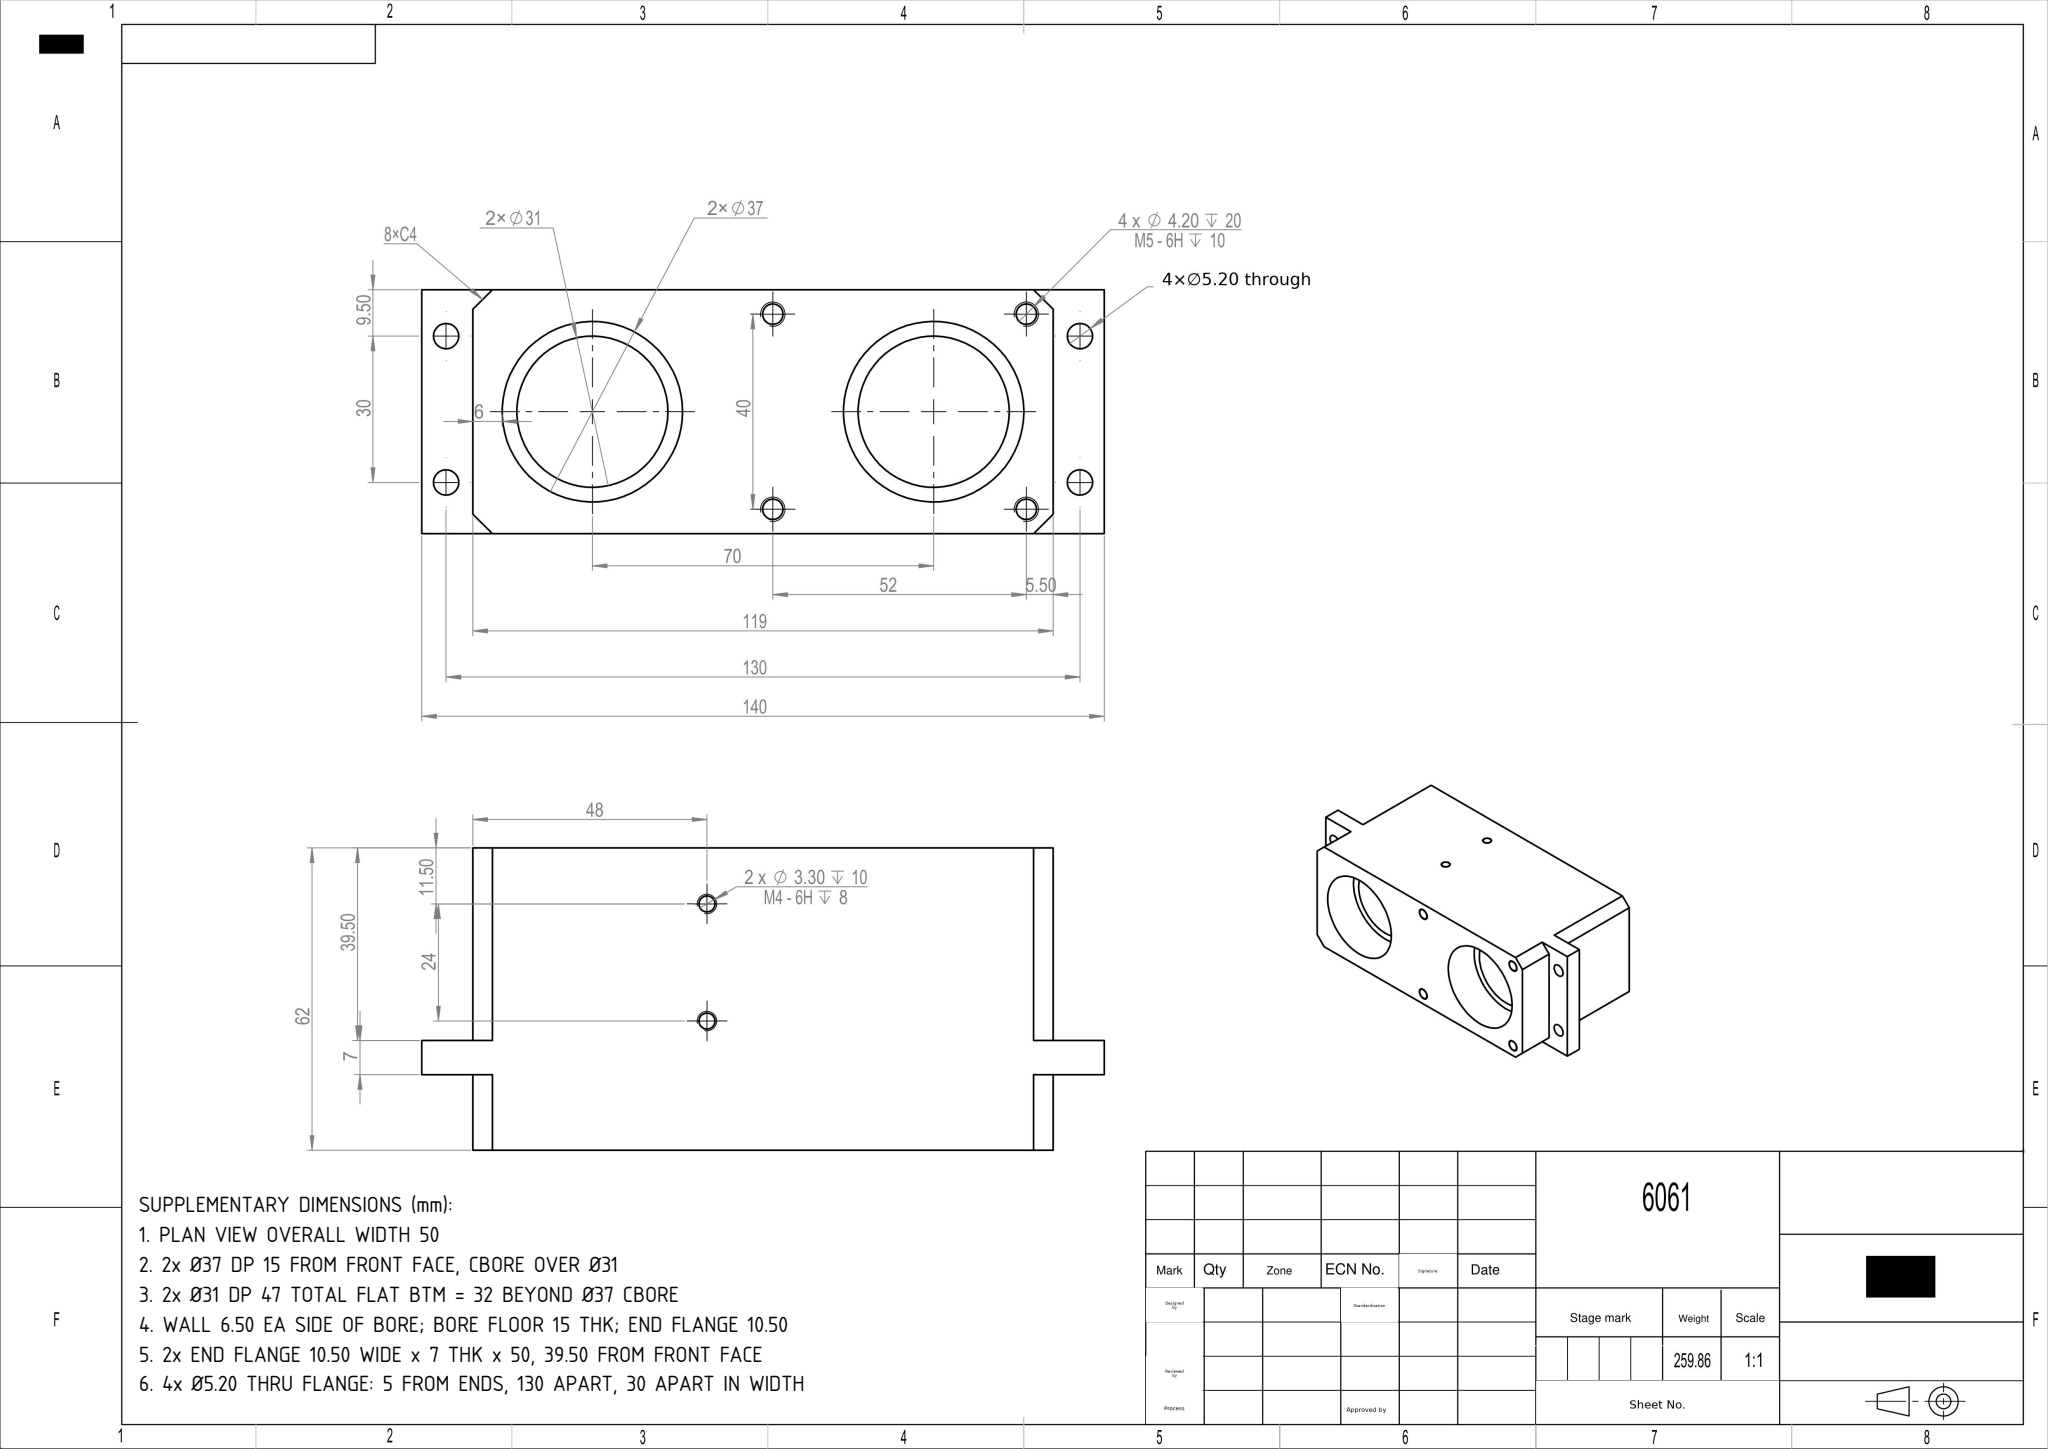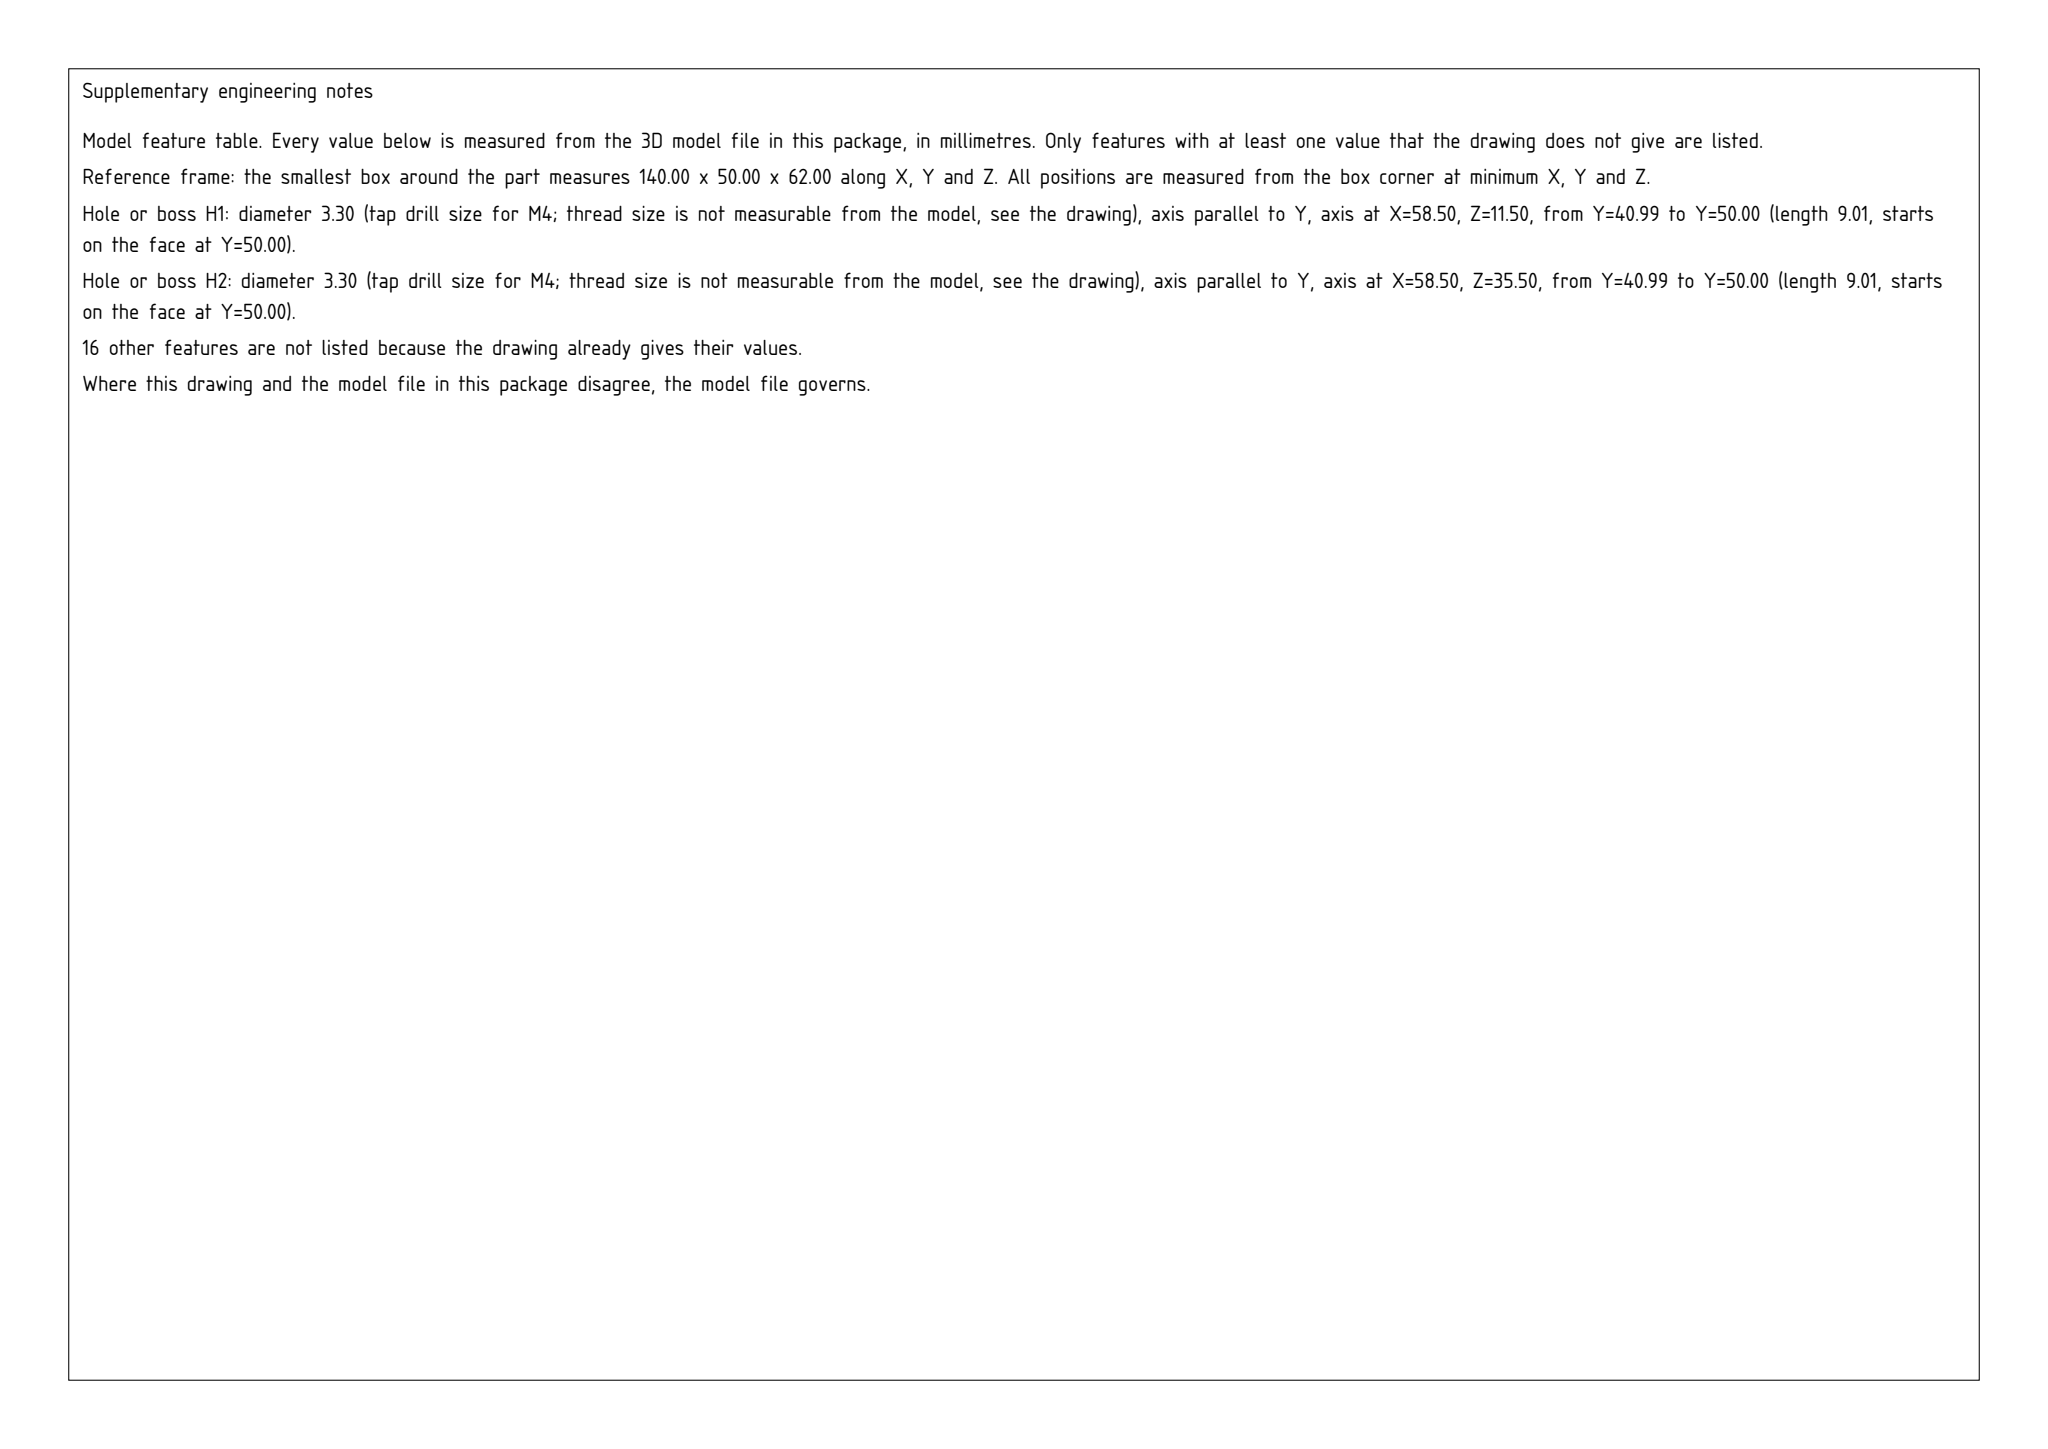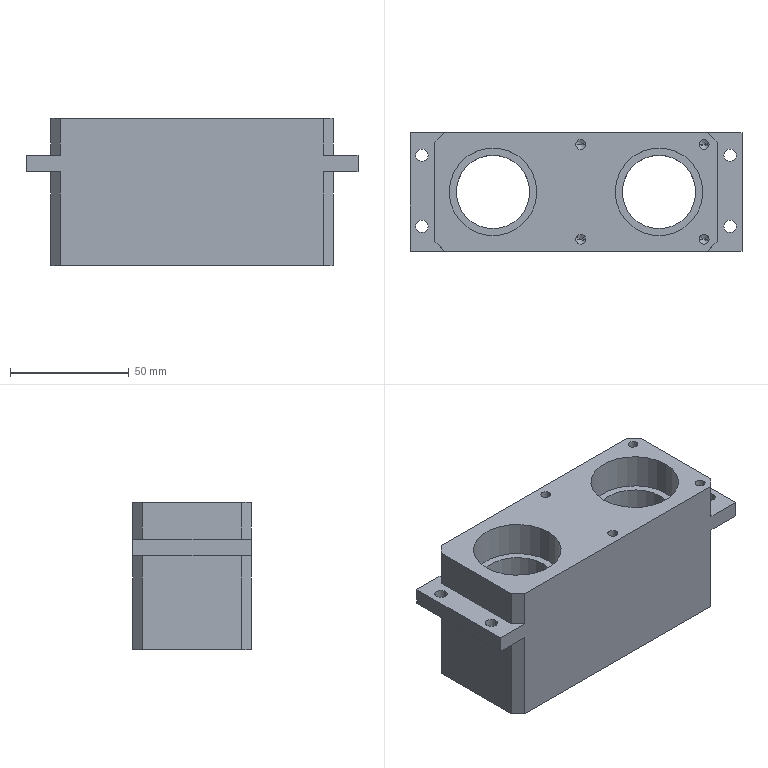Part | SolidWorks | mm | 1 solid | 70 faces | box 140 x 50 x 62 mm | volume 259856 mm3 | cylinder 32 | plane 26 | cone 12 | commonest cylinder face diameters 37 x8 4.2 x8 5.2 x8 3.3 x4 31 x4
build123d program:
from build123d import *

# Parameters (mm, degrees)
SKETCH1_W             = 119
SKETCH1_H             = 50
SKETCH1_R             = 15.5
BOSS_EXTRUDE1_DEPTH   = 62
SKETCH4_W             = 140
SKETCH4_H             = 50
SKETCH4_R             = 2.6
SKETCH4_R_2           = 15.5
BOSS_EXTRUDE2_DEPTH   = 7
CHAMFER2_SIZE         = 4
M5_TAPPED_HOLE1_D     = 4.2
M5_TAPPED_HOLE1_DEPTH = 18.738
M5_TAPPED_HOLE1_TIP   = 1.262
SKETCH8_R             = 18.5
CUT_EXTRUDE1_DEPTH    = 15
CUT_EXTRUDE2_START    = -15
SKETCH9_R             = 18.5
CUT_EXTRUDE2_DEPTH    = 15
M4_TAPPED_HOLE1_D     = 3.3
M4_TAPPED_HOLE1_DEPTH = 9.009
M4_TAPPED_HOLE1_TIP   = 0.9914


with BuildPart() as part:
    # Sketch1 → Boss-Extrude1 (new body)
    with BuildSketch(Plane.XY):
        Rectangle(SKETCH1_W, SKETCH1_H)
        with Locations((-35, 0)):
            Circle(SKETCH1_R, mode=Mode.SUBTRACT)
        with Locations((35, 0)):
            Circle(SKETCH1_R, mode=Mode.SUBTRACT)
    extrude(amount=BOSS_EXTRUDE1_DEPTH)

    # Sketch4 → Boss-Extrude2 (add)
    with BuildSketch(Plane(origin=(0, 0, 39.5), x_dir=(-1, 0, 0), z_dir=(0, 0, -1))):
        Rectangle(SKETCH4_W, SKETCH4_H)
        with Locations((-65, 15.5)):
            Circle(SKETCH4_R, mode=Mode.SUBTRACT)
        with Locations((65, 15.5)):
            Circle(SKETCH4_R, mode=Mode.SUBTRACT)
        with Locations((65, -14.5)):
            Circle(SKETCH4_R, mode=Mode.SUBTRACT)
        with Locations((-65, -14.5)):
            Circle(SKETCH4_R, mode=Mode.SUBTRACT)
        with Locations(Location((35, 0, 0), (0, 0, 180))):
            Circle(SKETCH4_R_2, mode=Mode.SUBTRACT)
        with Locations(Location((-35, 0, 0), (0, 0, 180))):
            Circle(SKETCH4_R_2, mode=Mode.SUBTRACT)
    extrude(amount=-BOSS_EXTRUDE2_DEPTH)

    # Chamfer2
    chamfer2_edges = [part.edges().sort_by_distance(p)[0] for p in [
        (59.5, -25, 19.75),
        (-59.5, -25, 19.75),
        (-59.5, 25, 19.75),
        (59.5, 25, 19.75),
        (59.5, -25, 54.25),
        (-59.5, -25, 54.25),
        (-59.5, 25, 54.25),
        (59.5, 25, 54.25),
    ]]
    chamfer(chamfer2_edges, length=CHAMFER2_SIZE)

    # M5 Tapped Hole1
    with Locations(Plane(origin=(0, 0, 62), x_dir=(-1, 0, 0), z_dir=(0, 0, 1))):
        with Locations((-54, -20), (-2, -20), (-2, 20), (-54, 20)):
            Hole(M5_TAPPED_HOLE1_D / 2, depth=M5_TAPPED_HOLE1_DEPTH)
            with Locations((0, 0, -(M5_TAPPED_HOLE1_DEPTH + M5_TAPPED_HOLE1_TIP / 2))):  # 118° drill point
                Cone(0, M5_TAPPED_HOLE1_D / 2, M5_TAPPED_HOLE1_TIP, mode=Mode.SUBTRACT)

    # Sketch8 → Cut-Extrude1 (cut)
    with BuildSketch(Plane(origin=(0, 0, 0), x_dir=(-1, 0, 0), z_dir=(0, 0, -1))):
        with Locations((-35, 0)):
            Circle(SKETCH8_R)
    cut_extrude1 = extrude(amount=-CUT_EXTRUDE1_DEPTH, mode=Mode.SUBTRACT)

    # Mirror1: Cut-Extrude1 across plane
    add(cut_extrude1.mirror(Plane(origin=(0, 0, 0), x_dir=(0, 0, 1), z_dir=(1, 0, 0))), mode=Mode.SUBTRACT)

    # Sketch9 → Cut-Extrude2 (cut)
    with BuildSketch(Plane.XY.offset(62).offset(CUT_EXTRUDE2_START)):
        with Locations((-35, 0)):
            Circle(SKETCH9_R)
        with Locations(Location((35, 0, 0), (0, 0, 180))):
            Circle(SKETCH9_R)
    extrude(amount=CUT_EXTRUDE2_DEPTH, mode=Mode.SUBTRACT)

    # M4 Tapped Hole1
    with Locations(Plane(origin=(0, 25, 0), x_dir=(1, 0, 0), z_dir=(0, 1, 0))):
        with Locations((-11.5, -11.5), (-11.5, -35.5)):
            Hole(M4_TAPPED_HOLE1_D / 2, depth=M4_TAPPED_HOLE1_DEPTH)
            with Locations((0, 0, -(M4_TAPPED_HOLE1_DEPTH + M4_TAPPED_HOLE1_TIP / 2))):  # 118° drill point
                Cone(0, M4_TAPPED_HOLE1_D / 2, M4_TAPPED_HOLE1_TIP, mode=Mode.SUBTRACT)


solid = part.part